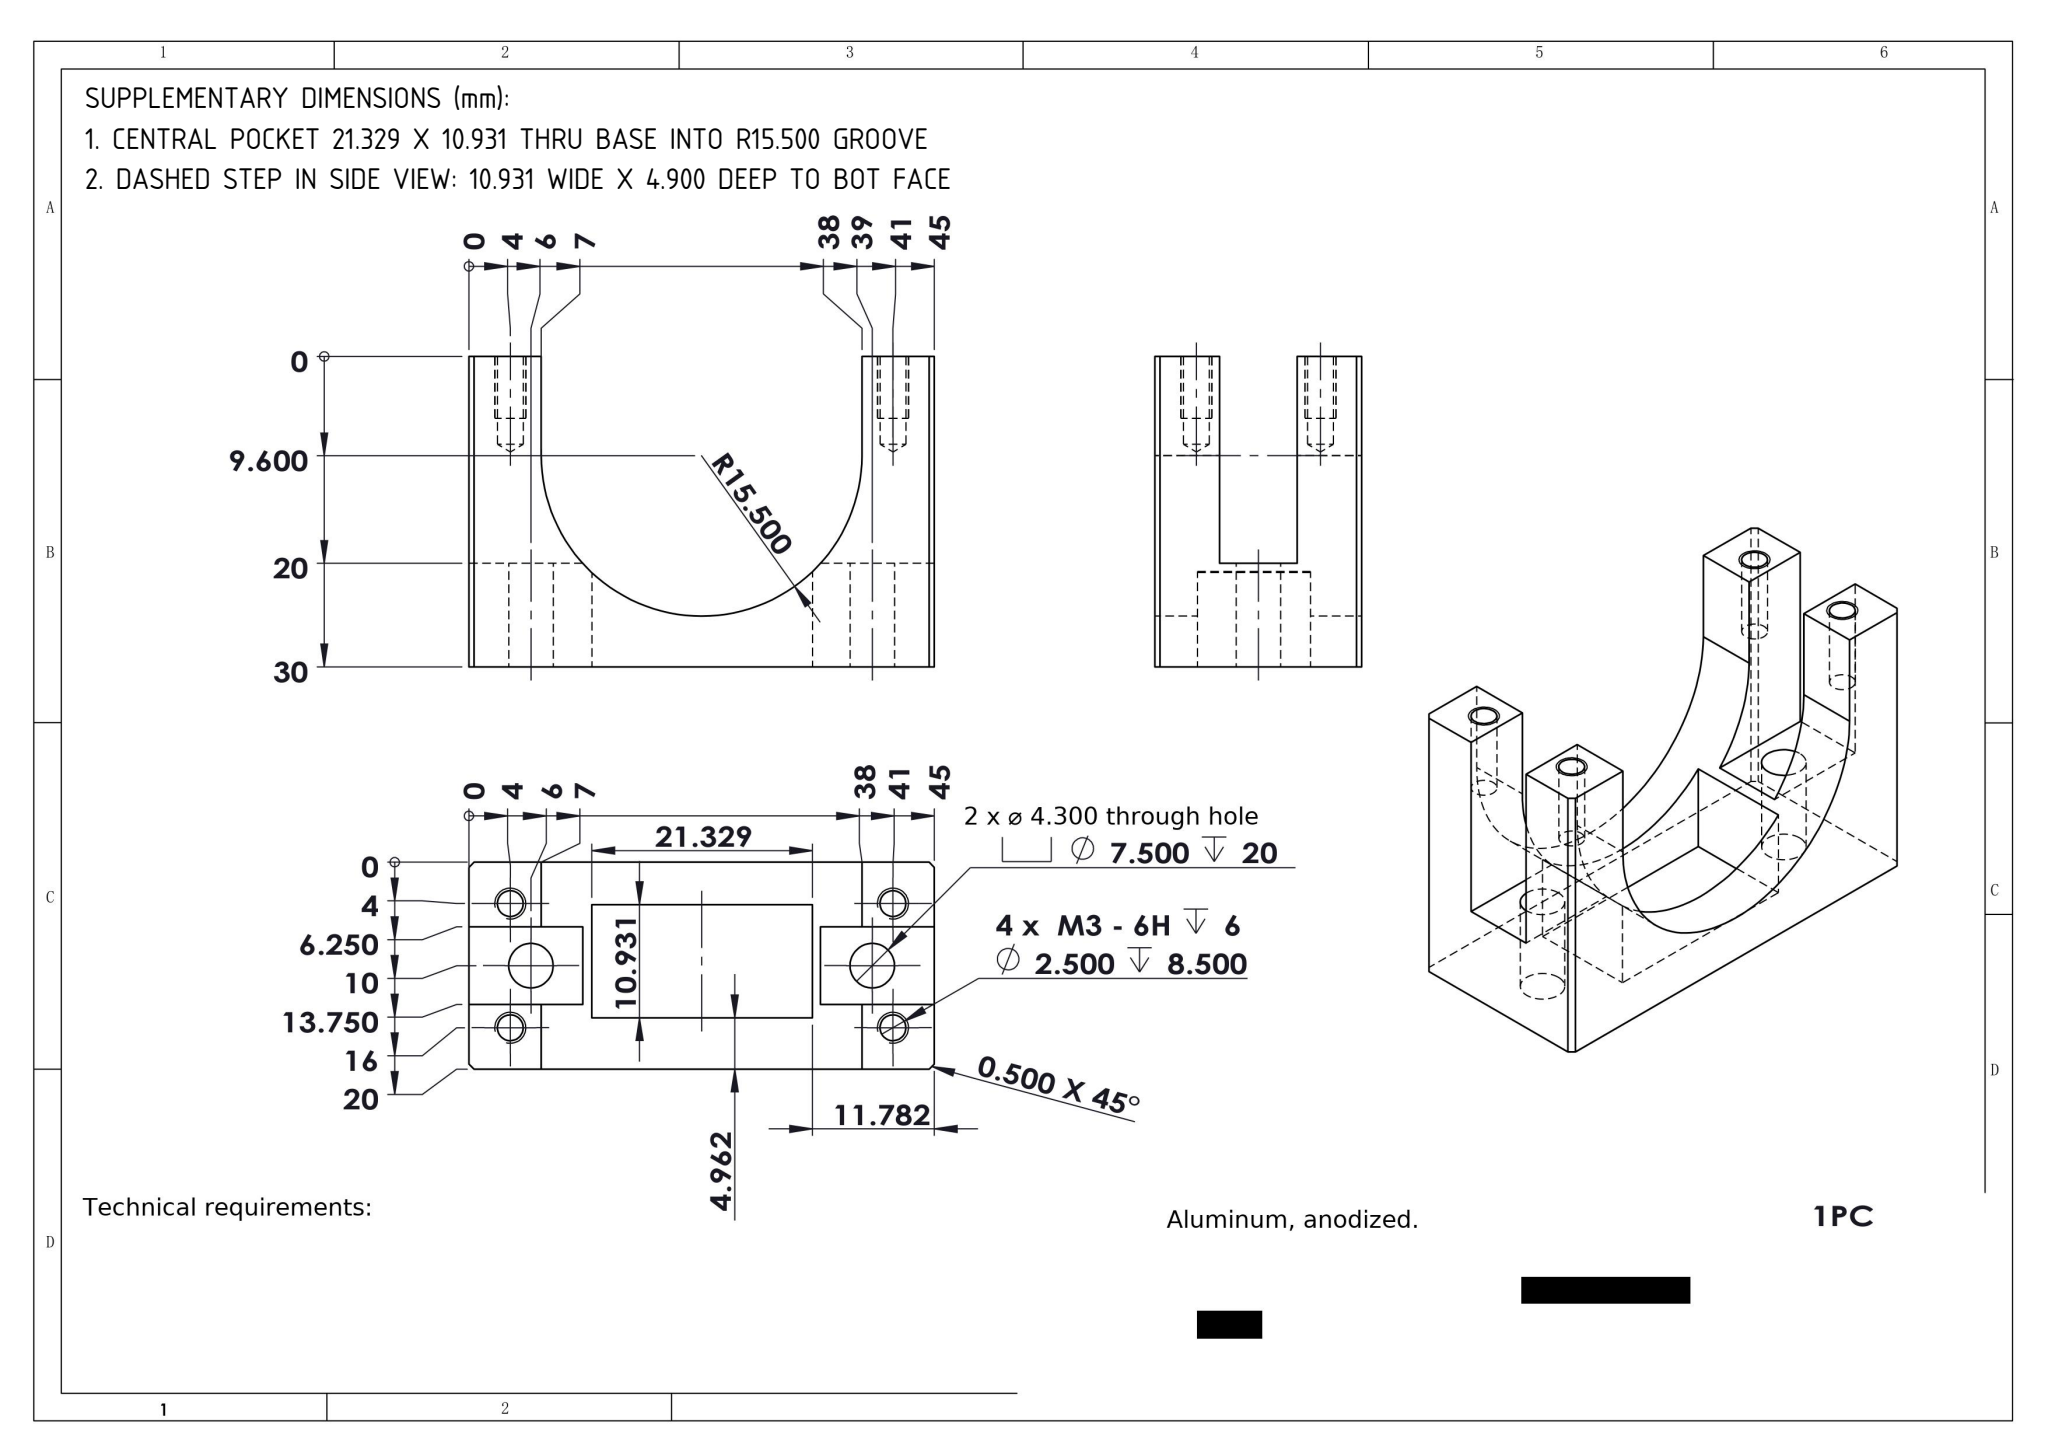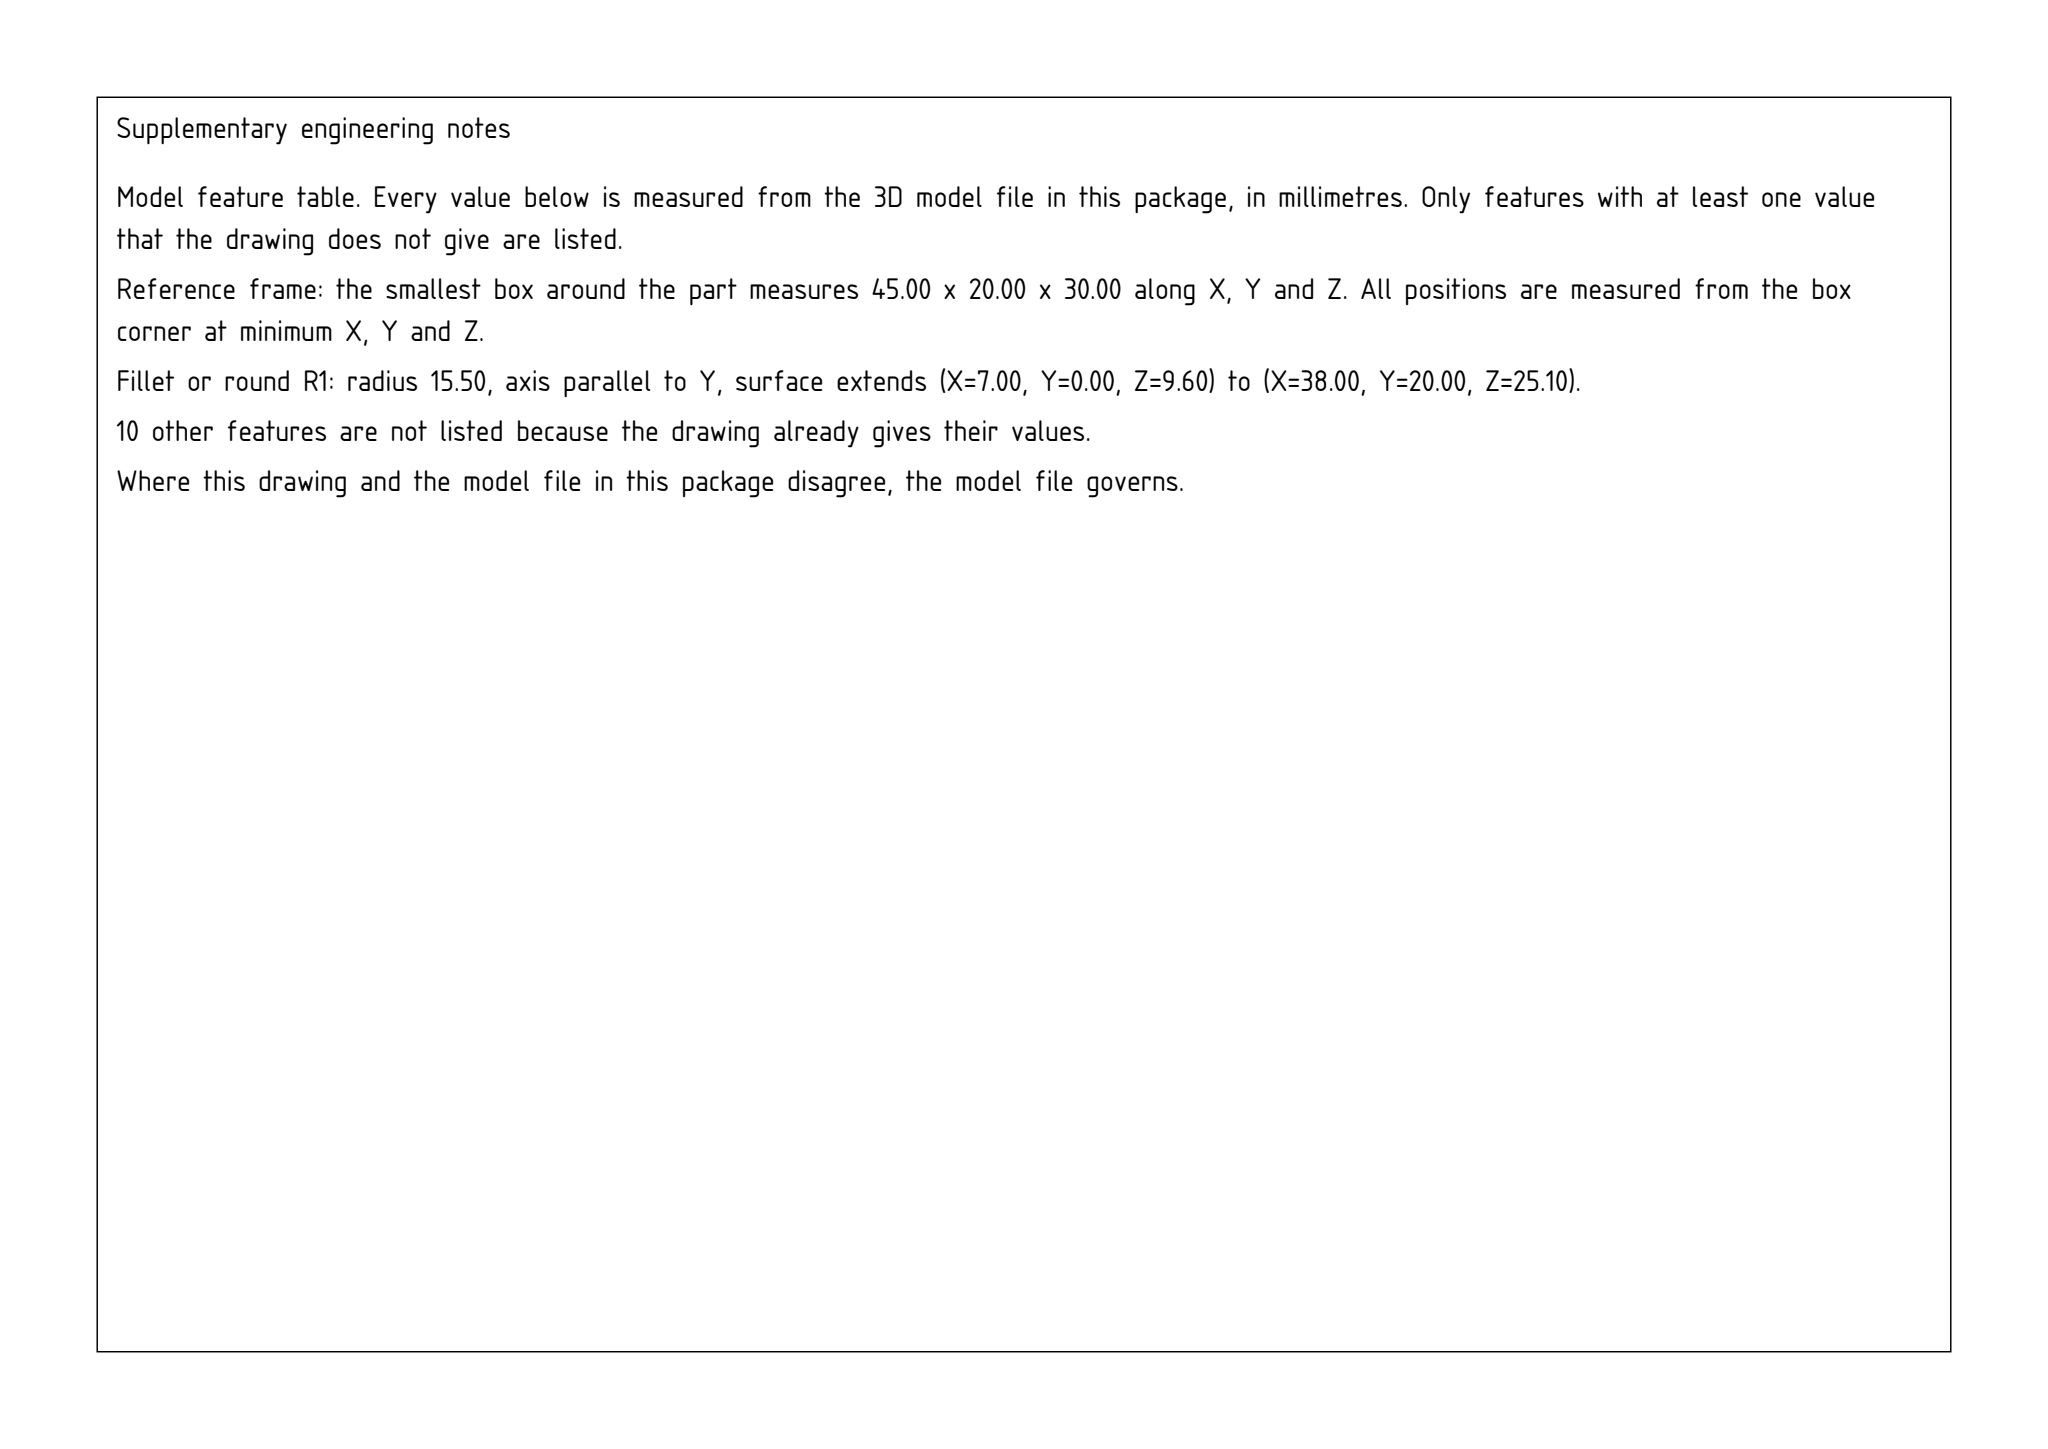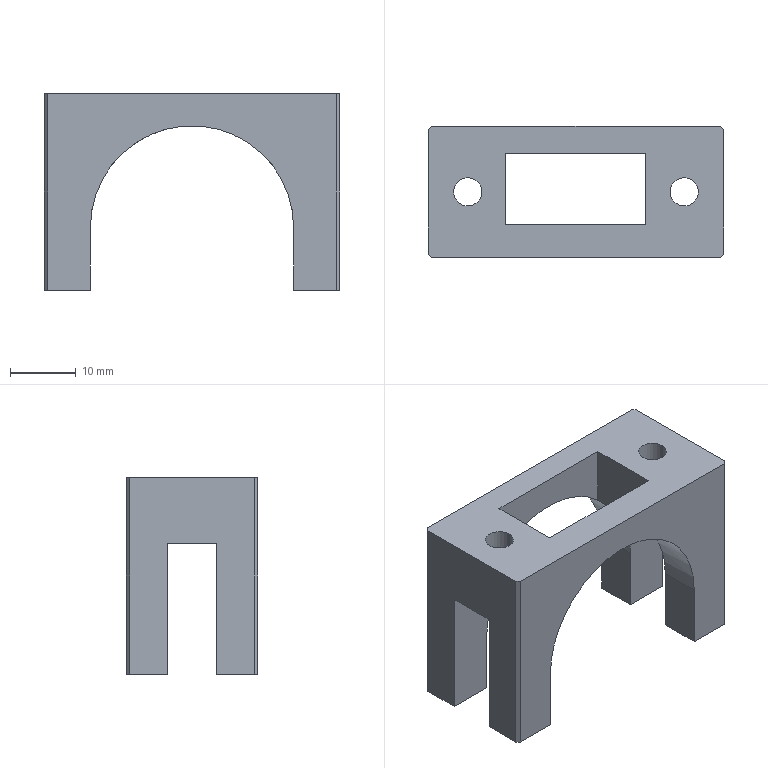Part | SolidWorks | mm | 1 solid | 48 faces | box 45 x 20 x 30 mm | volume 9274 mm3 | plane 27 | cylinder 13 | cone 8 | commonest cylinder face diameters 2.5 x8 4.3 x4 31 x1
build123d program:
from build123d import *

# Parameters (mm, degrees)
BOSS_EXTRUDE1_DEPTH                                  = 20
HOLE_SIZE_ACCORDING_TO_HEX_SOCKET_HEAD_C_D           = 4.3
HOLE_SIZE_ACCORDING_TO_HEX_SOCKET_HEAD_C_CBORE_D     = 7.5
HOLE_SIZE_ACCORDING_TO_HEX_SOCKET_HEAD_C_CBORE_DEPTH = 20
SKETCH6_W                                            = 45
SKETCH6_H                                            = 7.5
CUT_EXTRUDE1_DEPTH                                   = 32
M3_TAPPED_HOLE1_D                                    = 2.5
M3_TAPPED_HOLE1_DEPTH                                = 8.5
M3_TAPPED_HOLE1_TIP                                  = 0.7511
CHAMFER1_SIZE                                        = 0.5
SKETCH10_W                                           = 21.329
SKETCH10_H                                           = 10.931
CUT_EXTRUDE2_DEPTH                                   = 18


with BuildPart() as part:
    # Sketch1 → Boss-Extrude1 (new body)
    with BuildSketch(Plane(origin=(0, 0, 0), x_dir=(1, 0, 0), z_dir=(0, 1, 0))):
        with BuildLine():
            Line((38, 30), (45, 30))
            Line((45, 30), (45, 0))
            Line((45, 0), (0, 0))
            Line((0, 0), (0, 30))
            Line((0, 30), (7, 30))
            Line((7, 30), (7, 20.4))
            ThreePointArc((7, 20.4), (22.5, 4.9), (38, 20.4))
            Line((38, 20.4), (38, 30))
        make_face()
    extrude(amount=BOSS_EXTRUDE1_DEPTH)

    # Hole Size according to Hex Socket Head C (through all)
    with Locations(Plane(origin=(0, 0, -30), x_dir=(-1, 0, 0), z_dir=(0, 0, -1))):
        with Locations((-6, 10), (-39, 10)):
            CounterBoreHole(HOLE_SIZE_ACCORDING_TO_HEX_SOCKET_HEAD_C_D / 2, HOLE_SIZE_ACCORDING_TO_HEX_SOCKET_HEAD_C_CBORE_D / 2, HOLE_SIZE_ACCORDING_TO_HEX_SOCKET_HEAD_C_CBORE_DEPTH)

    # Sketch6 → Cut-Extrude1 (cut)
    with BuildSketch(Plane(origin=(0, 0, -10), x_dir=(-1, 0, 0), z_dir=(0, 0, -1))):
        with Locations((-22.5, 10)):
            Rectangle(SKETCH6_W, SKETCH6_H)
    extrude(amount=CUT_EXTRUDE1_DEPTH, mode=Mode.SUBTRACT)

    # M3 Tapped Hole1
    with Locations(Plane(origin=(0, 0, -30), x_dir=(-1, 0, 0), z_dir=(0, 0, -1))):
        with Locations((-41, 16), (-4, 16), (-4, 4), (-41, 4)):
            Hole(M3_TAPPED_HOLE1_D / 2, depth=M3_TAPPED_HOLE1_DEPTH)
            with Locations((0, 0, -(M3_TAPPED_HOLE1_DEPTH + M3_TAPPED_HOLE1_TIP / 2))):  # 118° drill point
                Cone(0, M3_TAPPED_HOLE1_D / 2, M3_TAPPED_HOLE1_TIP, mode=Mode.SUBTRACT)

    # Chamfer1
    chamfer1_edges = [part.edges().sort_by_distance(p)[0] for p in [
        (45, 20, -15),
        (0, 0, -15),
        (0, 20, -15),
        (45, 0, -15),
    ]]
    chamfer(chamfer1_edges, length=CHAMFER1_SIZE)

    # Sketch10 → Cut-Extrude2 (cut)
    with BuildSketch(Plane.XY):
        with Locations((22.447, 10.427)):
            Rectangle(SKETCH10_W, SKETCH10_H)
    extrude(amount=-CUT_EXTRUDE2_DEPTH, mode=Mode.SUBTRACT)


solid = part.part